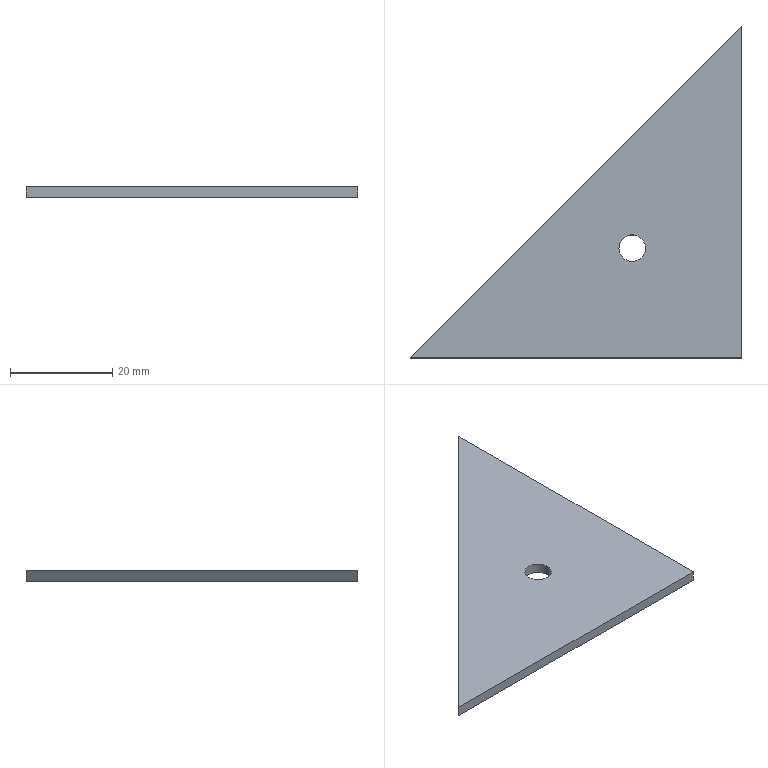Component | SolidWorks | SealingPlateAngleIron-3 | 1 solid | 7 faces | box 65 x 65 x 2 mm | volume 4183 mm3 | plane 5 | cylinder 2 | commonest cylinder face diameters 5.2 x2
build123d program:
from build123d import *

# Parameters (mm, degrees)
EXTRUDE1_DEPTH     = 2
CUT_EXTRUDE1_REACH = 93.946
SKETCH3_R          = 2.6


with BuildPart() as part:
    # Sketch1 → Extrude1 (new body)
    with BuildSketch(Plane.XY):
        Polygon((0, 0), (65, 0), (0, 65), align=None)
    extrude(amount=-EXTRUDE1_DEPTH)

    # Sketch3 → Cut-Extrude1 (cut, up to next)
    with BuildSketch(Plane(origin=(0, 0, -2), x_dir=(-1, 0, 0), z_dir=(0, 0, -1)), mode=Mode.PRIVATE) as cut_extrude1_sk1:
        with Locations((-21.5, 21.5)):
            Circle(SKETCH3_R)
    cut_extrude1_tool1 = extrude(cut_extrude1_sk1.sketch, amount=-CUT_EXTRUDE1_REACH, mode=Mode.PRIVATE) & part.part
    add(cut_extrude1_tool1.solids().sort_by_distance((21.5, 21.5, -2))[0], mode=Mode.SUBTRACT)


solid = part.part

# Placed as in the assembly
solid = solid.moved(Location((460, 100, -225.8), (0, 0, 90)))
STEP:
#1=COLOUR_RGB('',0.7922,0.8196,0.9333);
#2=FILL_AREA_STYLE_COLOUR('',#1);
#3=FILL_AREA_STYLE('',(#2));
#4=SURFACE_STYLE_FILL_AREA(#3);
#5=SURFACE_SIDE_STYLE('',(#4));
#6=SURFACE_STYLE_USAGE(.BOTH.,#5);
#7=PRESENTATION_STYLE_ASSIGNMENT((#6));
#8=CARTESIAN_POINT('',(17.161,4.783,-8.969));
#9=VERTEX_POINT('',#8);
#10=CARTESIAN_POINT('',(17.366,4.783,-8.969));
#11=VERTEX_POINT('',#10);
#12=CARTESIAN_POINT('',(17.264,4.783,-8.969));
#13=DIRECTION('',(0.,0.,1.));
#14=DIRECTION('',(-1.,0.,0.));
#15=AXIS2_PLACEMENT_3D('',#12,#13,#14);
#16=CIRCLE('',#15,0.1024);
#17=EDGE_CURVE('',#9,#11,#16,.T.);
#18=ORIENTED_EDGE('',*,*,#17,.F.);
#19=CARTESIAN_POINT('',(17.161,4.783,-8.89));
#20=VERTEX_POINT('',#19);
#21=CARTESIAN_POINT('',(17.161,4.783,-8.969));
#22=DIRECTION('',(0.,0.,1.));
#23=VECTOR('',#22,39.37);
#24=LINE('',#21,#23);
#25=EDGE_CURVE('',#9,#20,#24,.T.);
#26=ORIENTED_EDGE('',*,*,#25,.T.);
#27=CARTESIAN_POINT('',(17.366,4.783,-8.89));
#28=VERTEX_POINT('',#27);
#29=CARTESIAN_POINT('',(17.264,4.783,-8.89));
#30=DIRECTION('',(0.,0.,1.));
#31=DIRECTION('',(1.,0.,0.));
#32=AXIS2_PLACEMENT_3D('',#29,#30,#31);
#33=CIRCLE('',#32,0.1024);
#34=EDGE_CURVE('',#20,#28,#33,.T.);
#35=ORIENTED_EDGE('',*,*,#34,.T.);
#36=CARTESIAN_POINT('',(17.366,4.783,-8.969));
#37=DIRECTION('',(0.,0.,1.));
#38=VECTOR('',#37,39.37);
#39=LINE('',#36,#38);
#40=EDGE_CURVE('',#11,#28,#39,.T.);
#41=ORIENTED_EDGE('',*,*,#40,.F.);
#42=EDGE_LOOP('',(#18,#26,#35,#41));
#43=FACE_OUTER_BOUND('',#42,.T.);
#44=CARTESIAN_POINT('',(17.264,4.783,-8.969));
#45=DIRECTION('',(0.,0.,1.));
#46=DIRECTION('',(1.,0.,0.));
#47=AXIS2_PLACEMENT_3D('',#44,#45,#46);
#48=CYLINDRICAL_SURFACE('',#47,0.1024);
#49=ADVANCED_FACE('',(#43),#48,.F.);
#50=CARTESIAN_POINT('',(18.11,6.496,-8.969));
#51=VERTEX_POINT('',#50);
#52=CARTESIAN_POINT('',(18.11,3.937,-8.969));
#53=VERTEX_POINT('',#52);
#54=CARTESIAN_POINT('',(18.11,6.496,-8.969));
#55=DIRECTION('',(-0.,-1.,0.));
#56=VECTOR('',#55,39.37);
#57=LINE('',#54,#56);
#58=EDGE_CURVE('',#51,#53,#57,.T.);
#59=ORIENTED_EDGE('',*,*,#58,.F.);
#60=CARTESIAN_POINT('',(18.11,6.496,-8.89));
#61=VERTEX_POINT('',#60);
#62=CARTESIAN_POINT('',(18.11,6.496,-8.89));
#63=DIRECTION('',(0.,0.,-1.));
#64=VECTOR('',#63,39.37);
#65=LINE('',#62,#64);
#66=EDGE_CURVE('',#61,#51,#65,.T.);
#67=ORIENTED_EDGE('',*,*,#66,.F.);
#68=CARTESIAN_POINT('',(18.11,3.937,-8.89));
#69=VERTEX_POINT('',#68);
#70=CARTESIAN_POINT('',(18.11,6.496,-8.89));
#71=DIRECTION('',(-0.,-1.,0.));
#72=VECTOR('',#71,39.37);
#73=LINE('',#70,#72);
#74=EDGE_CURVE('',#61,#69,#73,.T.);
#75=ORIENTED_EDGE('',*,*,#74,.T.);
#76=CARTESIAN_POINT('',(18.11,3.937,-8.89));
#77=DIRECTION('',(0.,0.,-1.));
#78=VECTOR('',#77,39.37);
#79=LINE('',#76,#78);
#80=EDGE_CURVE('',#69,#53,#79,.T.);
#81=ORIENTED_EDGE('',*,*,#80,.T.);
#82=EDGE_LOOP('',(#59,#67,#75,#81));
#83=FACE_OUTER_BOUND('',#82,.T.);
#84=CARTESIAN_POINT('',(18.11,6.496,-8.89));
#85=DIRECTION('',(1.,-0.,0.));
#86=DIRECTION('',(-0.,-1.,0.));
#87=AXIS2_PLACEMENT_3D('',#84,#85,#86);
#88=PLANE('',#87);
#89=ADVANCED_FACE('',(#83),#88,.T.);
#90=CARTESIAN_POINT('',(15.551,3.937,-8.969));
#91=VERTEX_POINT('',#90);
#92=CARTESIAN_POINT('',(15.551,3.937,-8.969));
#93=DIRECTION('',(0.7071,0.7071,0.));
#94=VECTOR('',#93,39.37);
#95=LINE('',#92,#94);
#96=EDGE_CURVE('',#91,#51,#95,.T.);
#97=ORIENTED_EDGE('',*,*,#96,.F.);
#98=CARTESIAN_POINT('',(15.551,3.937,-8.89));
#99=VERTEX_POINT('',#98);
#100=CARTESIAN_POINT('',(15.551,3.937,-8.89));
#101=DIRECTION('',(0.,0.,-1.));
#102=VECTOR('',#101,39.37);
#103=LINE('',#100,#102);
#104=EDGE_CURVE('',#99,#91,#103,.T.);
#105=ORIENTED_EDGE('',*,*,#104,.F.);
#106=CARTESIAN_POINT('',(15.551,3.937,-8.89));
#107=DIRECTION('',(0.7071,0.7071,0.));
#108=VECTOR('',#107,39.37);
#109=LINE('',#106,#108);
#110=EDGE_CURVE('',#99,#61,#109,.T.);
#111=ORIENTED_EDGE('',*,*,#110,.T.);
#112=ORIENTED_EDGE('',*,*,#66,.T.);
#113=EDGE_LOOP('',(#97,#105,#111,#112));
#114=FACE_OUTER_BOUND('',#113,.T.);
#115=CARTESIAN_POINT('',(15.551,3.937,-8.89));
#116=DIRECTION('',(-0.7071,0.7071,0.));
#117=DIRECTION('',(0.7071,0.7071,0.));
#118=AXIS2_PLACEMENT_3D('',#115,#116,#117);
#119=PLANE('',#118);
#120=ADVANCED_FACE('',(#114),#119,.T.);
#121=CARTESIAN_POINT('',(18.11,3.937,-8.969));
#122=DIRECTION('',(-1.,0.,0.));
#123=VECTOR('',#122,39.37);
#124=LINE('',#121,#123);
#125=EDGE_CURVE('',#53,#91,#124,.T.);
#126=ORIENTED_EDGE('',*,*,#125,.F.);
#127=ORIENTED_EDGE('',*,*,#80,.F.);
#128=CARTESIAN_POINT('',(18.11,3.937,-8.89));
#129=DIRECTION('',(-1.,0.,0.));
#130=VECTOR('',#129,39.37);
#131=LINE('',#128,#130);
#132=EDGE_CURVE('',#69,#99,#131,.T.);
#133=ORIENTED_EDGE('',*,*,#132,.T.);
#134=ORIENTED_EDGE('',*,*,#104,.T.);
#135=EDGE_LOOP('',(#126,#127,#133,#134));
#136=FACE_OUTER_BOUND('',#135,.T.);
#137=CARTESIAN_POINT('',(18.11,3.937,-8.89));
#138=DIRECTION('',(0.,-1.,0.));
#139=DIRECTION('',(0.,0.,1.));
#140=AXIS2_PLACEMENT_3D('',#137,#138,#139);
#141=PLANE('',#140);
#142=ADVANCED_FACE('',(#136),#141,.T.);
#143=CARTESIAN_POINT('',(17.264,4.783,-8.89));
#144=DIRECTION('',(0.,0.,1.));
#145=DIRECTION('',(1.,0.,0.));
#146=AXIS2_PLACEMENT_3D('',#143,#144,#145);
#147=CIRCLE('',#146,0.1024);
#148=EDGE_CURVE('',#28,#20,#147,.T.);
#149=ORIENTED_EDGE('',*,*,#148,.F.);
#150=ORIENTED_EDGE('',*,*,#34,.F.);
#151=EDGE_LOOP('',(#149,#150));
#152=FACE_BOUND('',#151,.T.);
#153=ORIENTED_EDGE('',*,*,#74,.F.);
#154=ORIENTED_EDGE('',*,*,#110,.F.);
#155=ORIENTED_EDGE('',*,*,#132,.F.);
#156=EDGE_LOOP('',(#153,#154,#155));
#157=FACE_OUTER_BOUND('',#156,.T.);
#158=CARTESIAN_POINT('',(18.11,3.937,-8.89));
#159=DIRECTION('',(0.,0.,-1.));
#160=DIRECTION('',(-1.,0.,0.));
#161=AXIS2_PLACEMENT_3D('',#158,#159,#160);
#162=PLANE('',#161);
#163=ADVANCED_FACE('',(#152,#157),#162,.F.);
#164=CARTESIAN_POINT('',(17.264,4.783,-8.969));
#165=DIRECTION('',(0.,0.,1.));
#166=DIRECTION('',(-1.,0.,0.));
#167=AXIS2_PLACEMENT_3D('',#164,#165,#166);
#168=CIRCLE('',#167,0.1024);
#169=EDGE_CURVE('',#11,#9,#168,.T.);
#170=ORIENTED_EDGE('',*,*,#169,.T.);
#171=ORIENTED_EDGE('',*,*,#17,.T.);
#172=EDGE_LOOP('',(#170,#171));
#173=FACE_BOUND('',#172,.T.);
#174=ORIENTED_EDGE('',*,*,#58,.T.);
#175=ORIENTED_EDGE('',*,*,#125,.T.);
#176=ORIENTED_EDGE('',*,*,#96,.T.);
#177=EDGE_LOOP('',(#174,#175,#176));
#178=FACE_OUTER_BOUND('',#177,.T.);
#179=CARTESIAN_POINT('',(18.11,3.937,-8.969));
#180=DIRECTION('',(0.,0.,-1.));
#181=DIRECTION('',(-1.,0.,0.));
#182=AXIS2_PLACEMENT_3D('',#179,#180,#181);
#183=PLANE('',#182);
#184=ADVANCED_FACE('',(#173,#178),#183,.T.);
#185=ORIENTED_EDGE('',*,*,#25,.F.);
#186=ORIENTED_EDGE('',*,*,#169,.F.);
#187=ORIENTED_EDGE('',*,*,#40,.T.);
#188=ORIENTED_EDGE('',*,*,#148,.T.);
#189=EDGE_LOOP('',(#185,#186,#187,#188));
#190=FACE_OUTER_BOUND('',#189,.T.);
#191=CARTESIAN_POINT('',(17.264,4.783,-8.969));
#192=DIRECTION('',(0.,0.,1.));
#193=DIRECTION('',(1.,0.,0.));
#194=AXIS2_PLACEMENT_3D('',#191,#192,#193);
#195=CYLINDRICAL_SURFACE('',#194,0.1024);
#196=ADVANCED_FACE('',(#190),#195,.F.);
#197=CLOSED_SHELL('',(#49,#89,#120,#142,#163,#184,#196));
#198=MANIFOLD_SOLID_BREP('',#197);
#199=STYLED_ITEM('',(#7),#198);
#200=(LENGTH_UNIT()NAMED_UNIT(*)SI_UNIT($,.METRE.));
#201=LENGTH_MEASURE_WITH_UNIT(LENGTH_MEASURE(0.0254),#200);
#202=DIMENSIONAL_EXPONENTS(1.,0.,0.,0.,0.,0.,0.);
#203=(CONVERSION_BASED_UNIT('',#201)LENGTH_UNIT()NAMED_UNIT(#202));
#204=UNCERTAINTY_MEASURE_WITH_UNIT(LENGTH_MEASURE(0.00001),#203,'','');
#205=(NAMED_UNIT(*)PLANE_ANGLE_UNIT()SI_UNIT($,.RADIAN.));
#206=(NAMED_UNIT(*)SI_UNIT($,.STERADIAN.)SOLID_ANGLE_UNIT());
#207=(GEOMETRIC_REPRESENTATION_CONTEXT(3)GLOBAL_UNCERTAINTY_ASSIGNED_CONTEXT((#204))GLOBAL_UNIT_ASSIGNED_CONTEXT((#203,#205,#206))REPRESENTATION_CONTEXT('',''));
#208=MECHANICAL_DESIGN_GEOMETRIC_PRESENTATION_REPRESENTATION('',(#199),#207);
#209=CARTESIAN_POINT('',(0.,0.,0.));
#210=DIRECTION('',(0.,0.,1.));
#211=DIRECTION('',(1.,0.,0.));
#212=AXIS2_PLACEMENT_3D('',#209,#210,#211);
#213=(LENGTH_UNIT()NAMED_UNIT(*)SI_UNIT($,.METRE.));
#214=LENGTH_MEASURE_WITH_UNIT(LENGTH_MEASURE(0.0254),#213);
#215=DIMENSIONAL_EXPONENTS(1.,0.,0.,0.,0.,0.,0.);
#216=(CONVERSION_BASED_UNIT('',#214)LENGTH_UNIT()NAMED_UNIT(#215));
#217=UNCERTAINTY_MEASURE_WITH_UNIT(LENGTH_MEASURE(0.00001),#216,'','');
#218=(NAMED_UNIT(*)PLANE_ANGLE_UNIT()SI_UNIT($,.RADIAN.));
#219=(NAMED_UNIT(*)SI_UNIT($,.STERADIAN.)SOLID_ANGLE_UNIT());
#220=(GEOMETRIC_REPRESENTATION_CONTEXT(3)GLOBAL_UNCERTAINTY_ASSIGNED_CONTEXT((#217))GLOBAL_UNIT_ASSIGNED_CONTEXT((#216,#218,#219))REPRESENTATION_CONTEXT('',''));
#221=ADVANCED_BREP_SHAPE_REPRESENTATION('',(#198,#212),#220);
#222=PRESENTATION_LAYER_ASSIGNMENT('','',(#199));